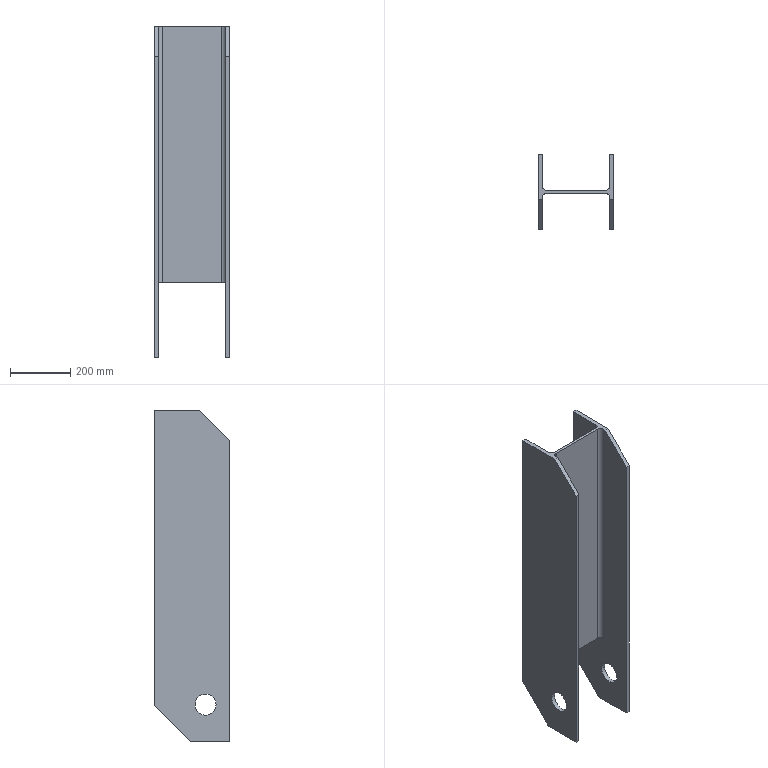Component | SolidWorks | WeldedI-beam-1_250I-beam-1 | 1 solid | 26 faces | box 250 x 250 x 1100 mm | volume 9072254 mm3 | plane 18 | cylinder 8 | commonest cylinder face diameters 70 x4 26 x4 | material Plain Carbon Steel
build123d program:
from build123d import *

# Parameters (mm, degrees)
BOSS_EXTRUDE1_DEPTH = 1100
SKETCH2_W           = 222
SKETCH2_H           = 250
CUT_EXTRUDE1_DEPTH  = 1156.422
CHAMFER1_SIZE       = 100
CHAMFER2_SIZE       = 120
SKETCH3_R           = 35
CUT_EXTRUDE2_DEPTH  = 1156.422


with BuildPart() as part:
    # Sketch1 → Boss-Extrude1 (new body)
    with BuildSketch(Plane(origin=(0, 0, 0), x_dir=(1, 0, 0), z_dir=(0, 1, 0))):
        with BuildLine():
            Line((0, 0), (250, 0))
            Line((250, 0), (250, -14))
            Line((250, -14), (142.5, -14))
            ThreePointArc((142.5, -14), (133.308, -17.808), (129.5, -27))
            Line((129.5, -27), (129.5, -223))
            ThreePointArc((129.5, -223), (133.308, -232.192), (142.5, -236))
            Line((142.5, -236), (250, -236))
            Line((250, -236), (250, -250))
            Line((250, -250), (0, -250))
            Line((0, -250), (0, -236))
            Line((0, -236), (107.5, -236))
            ThreePointArc((107.5, -236), (116.692, -232.192), (120.5, -223))
            Line((120.5, -223), (120.5, -27))
            ThreePointArc((120.5, -27), (116.692, -17.808), (107.5, -14))
            Line((107.5, -14), (0, -14))
            Line((0, -14), (0, 0))
        make_face()
    extrude(amount=BOSS_EXTRUDE1_DEPTH)

    # Sketch2 → Cut-Extrude1 (cut, through all)
    with BuildSketch(Plane.ZY):
        with Locations((125, 125)):
            Rectangle(SKETCH2_W, SKETCH2_H)
    extrude(amount=-CUT_EXTRUDE1_DEPTH, mode=Mode.SUBTRACT)

    # Chamfer1
    chamfer1_edges = [part.edges().sort_by_distance(p)[0] for p in [
        (250, 1100, 243),
        (250, 1100, 7),
    ]]
    chamfer(chamfer1_edges, length=CHAMFER1_SIZE)

    # Chamfer2
    chamfer2_edges = [part.edges().sort_by_distance(p)[0] for p in [
        (0, 0, 243),
        (0, 0, 7),
    ]]
    chamfer(chamfer2_edges, length=CHAMFER2_SIZE)

    # Sketch3 → Cut-Extrude2 (cut, through all)
    with BuildSketch(Plane.XY.offset(250)):
        with Locations((170, 123)):
            Circle(SKETCH3_R)
    extrude(amount=-CUT_EXTRUDE2_DEPTH, mode=Mode.SUBTRACT)


solid = part.part

# Placed as in the assembly
solid = solid.moved(Location((-6247.465, 2931.733, 5424.043), (90, -90, 0)))
STEP:
#1=CARTESIAN_POINT('',(-255.255,110.108,218.388));
#2=VERTEX_POINT('',#1);
#3=CARTESIAN_POINT('',(-255.255,107.352,218.388));
#4=VERTEX_POINT('',#3);
#5=CARTESIAN_POINT('',(-255.255,108.73,218.388));
#6=DIRECTION('',(-1.,-0.,0.));
#7=DIRECTION('',(0.,-1.,0.));
#8=AXIS2_PLACEMENT_3D('',#5,#6,#7);
#9=CIRCLE('',#8,1.378);
#10=EDGE_CURVE('',#2,#4,#9,.T.);
#11=ORIENTED_EDGE('',*,*,#10,.F.);
#12=CARTESIAN_POINT('',(-255.806,110.108,218.388));
#13=VERTEX_POINT('',#12);
#14=CARTESIAN_POINT('',(-245.963,110.108,218.388));
#15=DIRECTION('',(-1.,-0.,0.));
#16=VECTOR('',#15,39.37);
#17=LINE('',#14,#16);
#18=EDGE_CURVE('',#2,#13,#17,.T.);
#19=ORIENTED_EDGE('',*,*,#18,.T.);
#20=CARTESIAN_POINT('',(-255.806,107.352,218.388));
#21=VERTEX_POINT('',#20);
#22=CARTESIAN_POINT('',(-255.806,108.73,218.388));
#23=DIRECTION('',(-1.,-0.,0.));
#24=DIRECTION('',(0.,-1.,0.));
#25=AXIS2_PLACEMENT_3D('',#22,#23,#24);
#26=CIRCLE('',#25,1.378);
#27=EDGE_CURVE('',#13,#21,#26,.T.);
#28=ORIENTED_EDGE('',*,*,#27,.T.);
#29=CARTESIAN_POINT('',(-245.963,107.352,218.388));
#30=DIRECTION('',(-1.,-0.,0.));
#31=VECTOR('',#30,39.37);
#32=LINE('',#29,#31);
#33=EDGE_CURVE('',#4,#21,#32,.T.);
#34=ORIENTED_EDGE('',*,*,#33,.F.);
#35=EDGE_LOOP('',(#11,#19,#28,#34));
#36=FACE_OUTER_BOUND('',#35,.T.);
#37=CARTESIAN_POINT('',(-245.963,108.73,218.388));
#38=DIRECTION('',(-1.,-0.,0.));
#39=DIRECTION('',(0.,-1.,0.));
#40=AXIS2_PLACEMENT_3D('',#37,#38,#39);
#41=CYLINDRICAL_SURFACE('',#40,1.378);
#42=ADVANCED_FACE('',(#36),#41,.F.);
#43=CARTESIAN_POINT('',(-245.963,110.108,218.388));
#44=VERTEX_POINT('',#43);
#45=CARTESIAN_POINT('',(-245.963,107.352,218.388));
#46=VERTEX_POINT('',#45);
#47=CARTESIAN_POINT('',(-245.963,108.73,218.388));
#48=DIRECTION('',(-1.,-0.,0.));
#49=DIRECTION('',(0.,-1.,0.));
#50=AXIS2_PLACEMENT_3D('',#47,#48,#49);
#51=CIRCLE('',#50,1.378);
#52=EDGE_CURVE('',#44,#46,#51,.T.);
#53=ORIENTED_EDGE('',*,*,#52,.F.);
#54=CARTESIAN_POINT('',(-246.514,110.108,218.388));
#55=VERTEX_POINT('',#54);
#56=CARTESIAN_POINT('',(-245.963,110.108,218.388));
#57=DIRECTION('',(-1.,-0.,0.));
#58=VECTOR('',#57,39.37);
#59=LINE('',#56,#58);
#60=EDGE_CURVE('',#44,#55,#59,.T.);
#61=ORIENTED_EDGE('',*,*,#60,.T.);
#62=CARTESIAN_POINT('',(-246.514,107.352,218.388));
#63=VERTEX_POINT('',#62);
#64=CARTESIAN_POINT('',(-246.514,108.73,218.388));
#65=DIRECTION('',(1.,0.,-0.));
#66=DIRECTION('',(0.,1.,0.));
#67=AXIS2_PLACEMENT_3D('',#64,#65,#66);
#68=CIRCLE('',#67,1.378);
#69=EDGE_CURVE('',#63,#55,#68,.T.);
#70=ORIENTED_EDGE('',*,*,#69,.F.);
#71=CARTESIAN_POINT('',(-245.963,107.352,218.388));
#72=DIRECTION('',(-1.,-0.,0.));
#73=VECTOR('',#72,39.37);
#74=LINE('',#71,#73);
#75=EDGE_CURVE('',#46,#63,#74,.T.);
#76=ORIENTED_EDGE('',*,*,#75,.F.);
#77=EDGE_LOOP('',(#53,#61,#70,#76));
#78=FACE_OUTER_BOUND('',#77,.T.);
#79=CARTESIAN_POINT('',(-245.963,108.73,218.388));
#80=DIRECTION('',(-1.,-0.,0.));
#81=DIRECTION('',(0.,-1.,0.));
#82=AXIS2_PLACEMENT_3D('',#79,#80,#81);
#83=CYLINDRICAL_SURFACE('',#82,1.378);
#84=ADVANCED_FACE('',(#78),#83,.F.);
#85=CARTESIAN_POINT('',(-255.806,110.698,213.545));
#86=VERTEX_POINT('',#85);
#87=CARTESIAN_POINT('',(-255.806,105.58,213.545));
#88=VERTEX_POINT('',#87);
#89=CARTESIAN_POINT('',(-255.806,105.58,213.545));
#90=DIRECTION('',(0.,-1.,0.));
#91=VECTOR('',#90,39.37);
#92=LINE('',#89,#91);
#93=EDGE_CURVE('',#86,#88,#92,.T.);
#94=ORIENTED_EDGE('',*,*,#93,.F.);
#95=CARTESIAN_POINT('',(-255.255,110.698,213.545));
#96=VERTEX_POINT('',#95);
#97=CARTESIAN_POINT('',(-247.026,110.698,213.545));
#98=DIRECTION('',(1.,0.,-0.));
#99=VECTOR('',#98,39.37);
#100=LINE('',#97,#99);
#101=EDGE_CURVE('',#86,#96,#100,.T.);
#102=ORIENTED_EDGE('',*,*,#101,.T.);
#103=CARTESIAN_POINT('',(-255.255,105.58,213.545));
#104=VERTEX_POINT('',#103);
#105=CARTESIAN_POINT('',(-255.255,109.812,213.545));
#106=DIRECTION('',(-0.,1.,-0.));
#107=VECTOR('',#106,39.37);
#108=LINE('',#105,#107);
#109=EDGE_CURVE('',#104,#96,#108,.T.);
#110=ORIENTED_EDGE('',*,*,#109,.F.);
#111=CARTESIAN_POINT('',(-255.255,105.58,213.545));
#112=DIRECTION('',(1.,0.,-0.));
#113=VECTOR('',#112,39.37);
#114=LINE('',#111,#113);
#115=EDGE_CURVE('',#88,#104,#114,.T.);
#116=ORIENTED_EDGE('',*,*,#115,.F.);
#117=EDGE_LOOP('',(#94,#102,#110,#116));
#118=FACE_OUTER_BOUND('',#117,.T.);
#119=CARTESIAN_POINT('',(-247.026,109.812,213.545));
#120=DIRECTION('',(-0.,0.,1.));
#121=DIRECTION('',(-1.,-0.,0.));
#122=AXIS2_PLACEMENT_3D('',#119,#120,#121);
#123=PLANE('',#122);
#124=ADVANCED_FACE('',(#118),#123,.F.);
#125=CARTESIAN_POINT('',(-245.963,115.423,256.852));
#126=VERTEX_POINT('',#125);
#127=CARTESIAN_POINT('',(-245.963,115.423,218.269));
#128=VERTEX_POINT('',#127);
#129=CARTESIAN_POINT('',(-245.963,115.423,256.852));
#130=DIRECTION('',(0.,-0.,-1.));
#131=VECTOR('',#130,39.37);
#132=LINE('',#129,#131);
#133=EDGE_CURVE('',#126,#128,#132,.T.);
#134=ORIENTED_EDGE('',*,*,#133,.T.);
#135=CARTESIAN_POINT('',(-246.514,115.423,218.269));
#136=VERTEX_POINT('',#135);
#137=CARTESIAN_POINT('',(-246.514,115.423,218.269));
#138=DIRECTION('',(-1.,-0.,0.));
#139=VECTOR('',#138,39.37);
#140=LINE('',#137,#139);
#141=EDGE_CURVE('',#128,#136,#140,.T.);
#142=ORIENTED_EDGE('',*,*,#141,.T.);
#143=CARTESIAN_POINT('',(-246.514,115.423,256.852));
#144=VERTEX_POINT('',#143);
#145=CARTESIAN_POINT('',(-246.514,115.423,256.852));
#146=DIRECTION('',(0.,-0.,-1.));
#147=VECTOR('',#146,39.37);
#148=LINE('',#145,#147);
#149=EDGE_CURVE('',#144,#136,#148,.T.);
#150=ORIENTED_EDGE('',*,*,#149,.F.);
#151=CARTESIAN_POINT('',(-246.514,115.423,256.852));
#152=DIRECTION('',(-1.,-0.,0.));
#153=VECTOR('',#152,39.37);
#154=LINE('',#151,#153);
#155=EDGE_CURVE('',#126,#144,#154,.T.);
#156=ORIENTED_EDGE('',*,*,#155,.F.);
#157=EDGE_LOOP('',(#134,#142,#150,#156));
#158=FACE_OUTER_BOUND('',#157,.T.);
#159=CARTESIAN_POINT('',(-246.514,115.423,256.852));
#160=DIRECTION('',(0.,-1.,0.));
#161=DIRECTION('',(1.,0.,-0.));
#162=AXIS2_PLACEMENT_3D('',#159,#160,#161);
#163=PLANE('',#162);
#164=ADVANCED_FACE('',(#158),#163,.F.);
#165=CARTESIAN_POINT('',(-246.514,111.19,256.852));
#166=VERTEX_POINT('',#165);
#167=CARTESIAN_POINT('',(-246.514,111.19,223.388));
#168=VERTEX_POINT('',#167);
#169=CARTESIAN_POINT('',(-246.514,111.19,256.852));
#170=DIRECTION('',(0.,-0.,-1.));
#171=VECTOR('',#170,39.37);
#172=LINE('',#169,#171);
#173=EDGE_CURVE('',#166,#168,#172,.T.);
#174=ORIENTED_EDGE('',*,*,#173,.T.);
#175=CARTESIAN_POINT('',(-247.026,110.678,223.388));
#176=VERTEX_POINT('',#175);
#177=CARTESIAN_POINT('',(-247.026,111.19,223.388));
#178=DIRECTION('',(-0.,-0.,-1.));
#179=DIRECTION('',(-1.,0.,0.));
#180=AXIS2_PLACEMENT_3D('',#177,#178,#179);
#181=CIRCLE('',#180,0.5118);
#182=EDGE_CURVE('',#168,#176,#181,.T.);
#183=ORIENTED_EDGE('',*,*,#182,.T.);
#184=CARTESIAN_POINT('',(-247.026,110.678,256.852));
#185=VERTEX_POINT('',#184);
#186=CARTESIAN_POINT('',(-247.026,110.678,256.852));
#187=DIRECTION('',(0.,-0.,-1.));
#188=VECTOR('',#187,39.37);
#189=LINE('',#186,#188);
#190=EDGE_CURVE('',#185,#176,#189,.T.);
#191=ORIENTED_EDGE('',*,*,#190,.F.);
#192=CARTESIAN_POINT('',(-247.026,111.19,256.852));
#193=DIRECTION('',(0.,-0.,-1.));
#194=DIRECTION('',(1.,0.,0.));
#195=AXIS2_PLACEMENT_3D('',#192,#193,#194);
#196=CIRCLE('',#195,0.5118);
#197=EDGE_CURVE('',#166,#185,#196,.T.);
#198=ORIENTED_EDGE('',*,*,#197,.F.);
#199=EDGE_LOOP('',(#174,#183,#191,#198));
#200=FACE_OUTER_BOUND('',#199,.T.);
#201=CARTESIAN_POINT('',(-247.026,111.19,256.852));
#202=DIRECTION('',(0.,-0.,-1.));
#203=DIRECTION('',(1.,0.,0.));
#204=AXIS2_PLACEMENT_3D('',#201,#202,#203);
#205=CYLINDRICAL_SURFACE('',#204,0.5118);
#206=ADVANCED_FACE('',(#200),#205,.F.);
#207=ORIENTED_EDGE('',*,*,#190,.T.);
#208=CARTESIAN_POINT('',(-254.743,110.678,223.388));
#209=VERTEX_POINT('',#208);
#210=CARTESIAN_POINT('',(-254.743,110.678,223.388));
#211=DIRECTION('',(-1.,-0.,0.));
#212=VECTOR('',#211,39.37);
#213=LINE('',#210,#212);
#214=EDGE_CURVE('',#176,#209,#213,.T.);
#215=ORIENTED_EDGE('',*,*,#214,.T.);
#216=CARTESIAN_POINT('',(-254.743,110.678,256.852));
#217=VERTEX_POINT('',#216);
#218=CARTESIAN_POINT('',(-254.743,110.678,256.852));
#219=DIRECTION('',(0.,-0.,-1.));
#220=VECTOR('',#219,39.37);
#221=LINE('',#218,#220);
#222=EDGE_CURVE('',#217,#209,#221,.T.);
#223=ORIENTED_EDGE('',*,*,#222,.F.);
#224=CARTESIAN_POINT('',(-254.743,110.678,256.852));
#225=DIRECTION('',(-1.,-0.,0.));
#226=VECTOR('',#225,39.37);
#227=LINE('',#224,#226);
#228=EDGE_CURVE('',#185,#217,#227,.T.);
#229=ORIENTED_EDGE('',*,*,#228,.F.);
#230=EDGE_LOOP('',(#207,#215,#223,#229));
#231=FACE_OUTER_BOUND('',#230,.T.);
#232=CARTESIAN_POINT('',(-254.743,110.678,256.852));
#233=DIRECTION('',(0.,-1.,0.));
#234=DIRECTION('',(1.,0.,-0.));
#235=AXIS2_PLACEMENT_3D('',#232,#233,#234);
#236=PLANE('',#235);
#237=ADVANCED_FACE('',(#231),#236,.F.);
#238=ORIENTED_EDGE('',*,*,#222,.T.);
#239=CARTESIAN_POINT('',(-255.255,111.19,223.388));
#240=VERTEX_POINT('',#239);
#241=CARTESIAN_POINT('',(-254.743,111.19,223.388));
#242=DIRECTION('',(-0.,-0.,-1.));
#243=DIRECTION('',(-1.,-0.,0.));
#244=AXIS2_PLACEMENT_3D('',#241,#242,#243);
#245=CIRCLE('',#244,0.5118);
#246=EDGE_CURVE('',#209,#240,#245,.T.);
#247=ORIENTED_EDGE('',*,*,#246,.T.);
#248=CARTESIAN_POINT('',(-255.255,111.19,256.852));
#249=VERTEX_POINT('',#248);
#250=CARTESIAN_POINT('',(-255.255,111.19,256.852));
#251=DIRECTION('',(0.,-0.,-1.));
#252=VECTOR('',#251,39.37);
#253=LINE('',#250,#252);
#254=EDGE_CURVE('',#249,#240,#253,.T.);
#255=ORIENTED_EDGE('',*,*,#254,.F.);
#256=CARTESIAN_POINT('',(-254.743,111.19,256.852));
#257=DIRECTION('',(0.,-0.,-1.));
#258=DIRECTION('',(-1.,0.,0.));
#259=AXIS2_PLACEMENT_3D('',#256,#257,#258);
#260=CIRCLE('',#259,0.5118);
#261=EDGE_CURVE('',#217,#249,#260,.T.);
#262=ORIENTED_EDGE('',*,*,#261,.F.);
#263=EDGE_LOOP('',(#238,#247,#255,#262));
#264=FACE_OUTER_BOUND('',#263,.T.);
#265=CARTESIAN_POINT('',(-254.743,111.19,256.852));
#266=DIRECTION('',(0.,-0.,-1.));
#267=DIRECTION('',(1.,0.,0.));
#268=AXIS2_PLACEMENT_3D('',#265,#266,#267);
#269=CYLINDRICAL_SURFACE('',#268,0.5118);
#270=ADVANCED_FACE('',(#264),#269,.F.);
#271=CARTESIAN_POINT('',(-255.255,115.423,256.852));
#272=VERTEX_POINT('',#271);
#273=CARTESIAN_POINT('',(-255.255,115.423,218.269));
#274=VERTEX_POINT('',#273);
#275=CARTESIAN_POINT('',(-255.255,115.423,256.852));
#276=DIRECTION('',(0.,-0.,-1.));
#277=VECTOR('',#276,39.37);
#278=LINE('',#275,#277);
#279=EDGE_CURVE('',#272,#274,#278,.T.);
#280=ORIENTED_EDGE('',*,*,#279,.T.);
#281=CARTESIAN_POINT('',(-255.806,115.423,218.269));
#282=VERTEX_POINT('',#281);
#283=CARTESIAN_POINT('',(-255.806,115.423,218.269));
#284=DIRECTION('',(-1.,-0.,0.));
#285=VECTOR('',#284,39.37);
#286=LINE('',#283,#285);
#287=EDGE_CURVE('',#274,#282,#286,.T.);
#288=ORIENTED_EDGE('',*,*,#287,.T.);
#289=CARTESIAN_POINT('',(-255.806,115.423,256.852));
#290=VERTEX_POINT('',#289);
#291=CARTESIAN_POINT('',(-255.806,115.423,256.852));
#292=DIRECTION('',(0.,-0.,-1.));
#293=VECTOR('',#292,39.37);
#294=LINE('',#291,#293);
#295=EDGE_CURVE('',#290,#282,#294,.T.);
#296=ORIENTED_EDGE('',*,*,#295,.F.);
#297=CARTESIAN_POINT('',(-255.806,115.423,256.852));
#298=DIRECTION('',(-1.,-0.,0.));
#299=VECTOR('',#298,39.37);
#300=LINE('',#297,#299);
#301=EDGE_CURVE('',#272,#290,#300,.T.);
#302=ORIENTED_EDGE('',*,*,#301,.F.);
#303=EDGE_LOOP('',(#280,#288,#296,#302));
#304=FACE_OUTER_BOUND('',#303,.T.);
#305=CARTESIAN_POINT('',(-255.806,115.423,256.852));
#306=DIRECTION('',(0.,-1.,0.));
#307=DIRECTION('',(1.,0.,-0.));
#308=AXIS2_PLACEMENT_3D('',#305,#306,#307);
#309=PLANE('',#308);
#310=ADVANCED_FACE('',(#304),#309,.F.);
#311=CARTESIAN_POINT('',(-255.806,108.73,218.388));
#312=DIRECTION('',(-1.,-0.,0.));
#313=DIRECTION('',(0.,-1.,0.));
#314=AXIS2_PLACEMENT_3D('',#311,#312,#313);
#315=CIRCLE('',#314,1.378);
#316=EDGE_CURVE('',#21,#13,#315,.T.);
#317=ORIENTED_EDGE('',*,*,#316,.F.);
#318=ORIENTED_EDGE('',*,*,#27,.F.);
#319=EDGE_LOOP('',(#317,#318));
#320=FACE_BOUND('',#319,.T.);
#321=ORIENTED_EDGE('',*,*,#295,.T.);
#322=CARTESIAN_POINT('',(-255.806,115.423,218.269));
#323=DIRECTION('',(0.,-0.7071,-0.7071));
#324=VECTOR('',#323,39.37);
#325=LINE('',#322,#324);
#326=EDGE_CURVE('',#282,#86,#325,.T.);
#327=ORIENTED_EDGE('',*,*,#326,.T.);
#328=ORIENTED_EDGE('',*,*,#93,.T.);
#329=CARTESIAN_POINT('',(-255.806,105.58,252.915));
#330=VERTEX_POINT('',#329);
#331=CARTESIAN_POINT('',(-255.806,105.58,256.852));
#332=DIRECTION('',(0.,-0.,-1.));
#333=VECTOR('',#332,39.37);
#334=LINE('',#331,#333);
#335=EDGE_CURVE('',#330,#88,#334,.T.);
#336=ORIENTED_EDGE('',*,*,#335,.F.);
#337=CARTESIAN_POINT('',(-255.806,109.517,256.852));
#338=VERTEX_POINT('',#337);
#339=CARTESIAN_POINT('',(-255.806,109.517,256.852));
#340=DIRECTION('',(-0.,0.7071,0.7071));
#341=VECTOR('',#340,39.37);
#342=LINE('',#339,#341);
#343=EDGE_CURVE('',#330,#338,#342,.T.);
#344=ORIENTED_EDGE('',*,*,#343,.T.);
#345=CARTESIAN_POINT('',(-255.806,105.58,256.852));
#346=DIRECTION('',(0.,-1.,0.));
#347=VECTOR('',#346,39.37);
#348=LINE('',#345,#347);
#349=EDGE_CURVE('',#290,#338,#348,.T.);
#350=ORIENTED_EDGE('',*,*,#349,.F.);
#351=EDGE_LOOP('',(#321,#327,#328,#336,#344,#350));
#352=FACE_OUTER_BOUND('',#351,.T.);
#353=CARTESIAN_POINT('',(-255.806,105.58,256.852));
#354=DIRECTION('',(1.,0.,-0.));
#355=DIRECTION('',(-0.,1.,-0.));
#356=AXIS2_PLACEMENT_3D('',#353,#354,#355);
#357=PLANE('',#356);
#358=ADVANCED_FACE('',(#320,#352),#357,.F.);
#359=CARTESIAN_POINT('',(-255.255,105.58,252.915));
#360=VERTEX_POINT('',#359);
#361=CARTESIAN_POINT('',(-255.255,105.58,256.852));
#362=DIRECTION('',(0.,-0.,-1.));
#363=VECTOR('',#362,39.37);
#364=LINE('',#361,#363);
#365=EDGE_CURVE('',#360,#104,#364,.T.);
#366=ORIENTED_EDGE('',*,*,#365,.F.);
#367=CARTESIAN_POINT('',(-255.806,105.58,252.915));
#368=DIRECTION('',(-1.,-0.,0.));
#369=VECTOR('',#368,39.37);
#370=LINE('',#367,#369);
#371=EDGE_CURVE('',#360,#330,#370,.T.);
#372=ORIENTED_EDGE('',*,*,#371,.T.);
#373=ORIENTED_EDGE('',*,*,#335,.T.);
#374=ORIENTED_EDGE('',*,*,#115,.T.);
#375=EDGE_LOOP('',(#366,#372,#373,#374));
#376=FACE_OUTER_BOUND('',#375,.T.);
#377=CARTESIAN_POINT('',(-255.255,105.58,256.852));
#378=DIRECTION('',(-0.,1.,-0.));
#379=DIRECTION('',(-1.,-0.,0.));
#380=AXIS2_PLACEMENT_3D('',#377,#378,#379);
#381=PLANE('',#380);
#382=ADVANCED_FACE('',(#376),#381,.F.);
#383=CARTESIAN_POINT('',(-255.255,108.73,218.388));
#384=DIRECTION('',(-1.,-0.,0.));
#385=DIRECTION('',(0.,-1.,0.));
#386=AXIS2_PLACEMENT_3D('',#383,#384,#385);
#387=CIRCLE('',#386,1.378);
#388=EDGE_CURVE('',#4,#2,#387,.T.);
#389=ORIENTED_EDGE('',*,*,#388,.T.);
#390=ORIENTED_EDGE('',*,*,#10,.T.);
#391=EDGE_LOOP('',(#389,#390));
#392=FACE_BOUND('',#391,.T.);
#393=ORIENTED_EDGE('',*,*,#109,.T.);
#394=CARTESIAN_POINT('',(-255.255,115.423,218.269));
#395=DIRECTION('',(-0.,0.7071,0.7071));
#396=VECTOR('',#395,39.37);
#397=LINE('',#394,#396);
#398=EDGE_CURVE('',#96,#274,#397,.T.);
#399=ORIENTED_EDGE('',*,*,#398,.T.);
#400=ORIENTED_EDGE('',*,*,#279,.F.);
#401=CARTESIAN_POINT('',(-255.255,115.423,256.852));
#402=DIRECTION('',(-0.,1.,-0.));
#403=VECTOR('',#402,39.37);
#404=LINE('',#401,#403);
#405=EDGE_CURVE('',#249,#272,#404,.T.);
#406=ORIENTED_EDGE('',*,*,#405,.F.);
#407=ORIENTED_EDGE('',*,*,#254,.T.);
#408=CARTESIAN_POINT('',(-255.255,109.812,223.388));
#409=VERTEX_POINT('',#408);
#410=CARTESIAN_POINT('',(-255.255,105.58,223.388));
#411=DIRECTION('',(-0.,1.,-0.));
#412=VECTOR('',#411,39.37);
#413=LINE('',#410,#412);
#414=EDGE_CURVE('',#409,#240,#413,.T.);
#415=ORIENTED_EDGE('',*,*,#414,.F.);
#416=CARTESIAN_POINT('',(-255.255,109.812,256.852));
#417=VERTEX_POINT('',#416);
#418=CARTESIAN_POINT('',(-255.255,109.812,256.852));
#419=DIRECTION('',(0.,-0.,-1.));
#420=VECTOR('',#419,39.37);
#421=LINE('',#418,#420);
#422=EDGE_CURVE('',#417,#409,#421,.T.);
#423=ORIENTED_EDGE('',*,*,#422,.F.);
#424=CARTESIAN_POINT('',(-255.255,109.517,256.852));
#425=VERTEX_POINT('',#424);
#426=CARTESIAN_POINT('',(-255.255,109.812,256.852));
#427=DIRECTION('',(-0.,1.,-0.));
#428=VECTOR('',#427,39.37);
#429=LINE('',#426,#428);
#430=EDGE_CURVE('',#425,#417,#429,.T.);
#431=ORIENTED_EDGE('',*,*,#430,.F.);
#432=CARTESIAN_POINT('',(-255.255,109.517,256.852));
#433=DIRECTION('',(0.,-0.7071,-0.7071));
#434=VECTOR('',#433,39.37);
#435=LINE('',#432,#434);
#436=EDGE_CURVE('',#425,#360,#435,.T.);
#437=ORIENTED_EDGE('',*,*,#436,.T.);
#438=ORIENTED_EDGE('',*,*,#365,.T.);
#439=EDGE_LOOP('',(#393,#399,#400,#406,#407,#415,#423,#431,#437,#438));
#440=FACE_OUTER_BOUND('',#439,.T.);
#441=CARTESIAN_POINT('',(-255.255,109.812,256.852));
#442=DIRECTION('',(-1.,-0.,0.));
#443=DIRECTION('',(0.,-1.,0.));
#444=AXIS2_PLACEMENT_3D('',#441,#442,#443);
#445=PLANE('',#444);
#446=ADVANCED_FACE('',(#392,#440),#445,.F.);
#447=ORIENTED_EDGE('',*,*,#422,.T.);
#448=CARTESIAN_POINT('',(-254.743,110.324,223.388));
#449=VERTEX_POINT('',#448);
#450=CARTESIAN_POINT('',(-254.743,109.812,223.388));
#451=DIRECTION('',(-0.,-0.,-1.));
#452=DIRECTION('',(-1.,0.,0.));
#453=AXIS2_PLACEMENT_3D('',#450,#451,#452);
#454=CIRCLE('',#453,0.5118);
#455=EDGE_CURVE('',#409,#449,#454,.T.);
#456=ORIENTED_EDGE('',*,*,#455,.T.);
#457=CARTESIAN_POINT('',(-254.743,110.324,256.852));
#458=VERTEX_POINT('',#457);
#459=CARTESIAN_POINT('',(-254.743,110.324,256.852));
#460=DIRECTION('',(0.,-0.,-1.));
#461=VECTOR('',#460,39.37);
#462=LINE('',#459,#461);
#463=EDGE_CURVE('',#458,#449,#462,.T.);
#464=ORIENTED_EDGE('',*,*,#463,.F.);
#465=CARTESIAN_POINT('',(-254.743,109.812,256.852));
#466=DIRECTION('',(0.,-0.,-1.));
#467=DIRECTION('',(-1.,0.,0.));
#468=AXIS2_PLACEMENT_3D('',#465,#466,#467);
#469=CIRCLE('',#468,0.5118);
#470=EDGE_CURVE('',#417,#458,#469,.T.);
#471=ORIENTED_EDGE('',*,*,#470,.F.);
#472=EDGE_LOOP('',(#447,#456,#464,#471));
#473=FACE_OUTER_BOUND('',#472,.T.);
#474=CARTESIAN_POINT('',(-254.743,109.812,256.852));
#475=DIRECTION('',(0.,-0.,-1.));
#476=DIRECTION('',(1.,0.,0.));
#477=AXIS2_PLACEMENT_3D('',#474,#475,#476);
#478=CYLINDRICAL_SURFACE('',#477,0.5118);
#479=ADVANCED_FACE('',(#473),#478,.F.);
#480=ORIENTED_EDGE('',*,*,#463,.T.);
#481=CARTESIAN_POINT('',(-247.026,110.324,223.388));
#482=VERTEX_POINT('',#481);
#483=CARTESIAN_POINT('',(-247.026,110.324,223.388));
#484=DIRECTION('',(1.,0.,-0.));
#485=VECTOR('',#484,39.37);
#486=LINE('',#483,#485);
#487=EDGE_CURVE('',#449,#482,#486,.T.);
#488=ORIENTED_EDGE('',*,*,#487,.T.);
#489=CARTESIAN_POINT('',(-247.026,110.324,256.852));
#490=VERTEX_POINT('',#489);
#491=CARTESIAN_POINT('',(-247.026,110.324,256.852));
#492=DIRECTION('',(0.,-0.,-1.));
#493=VECTOR('',#492,39.37);
#494=LINE('',#491,#493);
#495=EDGE_CURVE('',#490,#482,#494,.T.);
#496=ORIENTED_EDGE('',*,*,#495,.F.);
#497=CARTESIAN_POINT('',(-247.026,110.324,256.852));
#498=DIRECTION('',(1.,0.,-0.));
#499=VECTOR('',#498,39.37);
#500=LINE('',#497,#499);
#501=EDGE_CURVE('',#458,#490,#500,.T.);
#502=ORIENTED_EDGE('',*,*,#501,.F.);
#503=EDGE_LOOP('',(#480,#488,#496,#502));
#504=FACE_OUTER_BOUND('',#503,.T.);
#505=CARTESIAN_POINT('',(-247.026,110.324,256.852));
#506=DIRECTION('',(-0.,1.,-0.));
#507=DIRECTION('',(-1.,-0.,0.));
#508=AXIS2_PLACEMENT_3D('',#505,#506,#507);
#509=PLANE('',#508);
#510=ADVANCED_FACE('',(#504),#509,.F.);
#511=ORIENTED_EDGE('',*,*,#495,.T.);
#512=CARTESIAN_POINT('',(-246.514,109.812,223.388));
#513=VERTEX_POINT('',#512);
#514=CARTESIAN_POINT('',(-247.026,109.812,223.388));
#515=DIRECTION('',(-0.,-0.,-1.));
#516=DIRECTION('',(-1.,0.,0.));
#517=AXIS2_PLACEMENT_3D('',#514,#515,#516);
#518=CIRCLE('',#517,0.5118);
#519=EDGE_CURVE('',#482,#513,#518,.T.);
#520=ORIENTED_EDGE('',*,*,#519,.T.);
#521=CARTESIAN_POINT('',(-246.514,109.812,256.852));
#522=VERTEX_POINT('',#521);
#523=CARTESIAN_POINT('',(-246.514,109.812,256.852));
#524=DIRECTION('',(0.,-0.,-1.));
#525=VECTOR('',#524,39.37);
#526=LINE('',#523,#525);
#527=EDGE_CURVE('',#522,#513,#526,.T.);
#528=ORIENTED_EDGE('',*,*,#527,.F.);
#529=CARTESIAN_POINT('',(-247.026,109.812,256.852));
#530=DIRECTION('',(0.,-0.,-1.));
#531=DIRECTION('',(-1.,0.,0.));
#532=AXIS2_PLACEMENT_3D('',#529,#530,#531);
#533=CIRCLE('',#532,0.5118);
#534=EDGE_CURVE('',#490,#522,#533,.T.);
#535=ORIENTED_EDGE('',*,*,#534,.F.);
#536=EDGE_LOOP('',(#511,#520,#528,#535));
#537=FACE_OUTER_BOUND('',#536,.T.);
#538=CARTESIAN_POINT('',(-247.026,109.812,256.852));
#539=DIRECTION('',(0.,-0.,-1.));
#540=DIRECTION('',(1.,0.,0.));
#541=AXIS2_PLACEMENT_3D('',#538,#539,#540);
#542=CYLINDRICAL_SURFACE('',#541,0.5118);
#543=ADVANCED_FACE('',(#537),#542,.F.);
#544=ORIENTED_EDGE('',*,*,#69,.T.);
#545=CARTESIAN_POINT('',(-246.514,108.73,218.388));
#546=DIRECTION('',(1.,0.,-0.));
#547=DIRECTION('',(0.,1.,0.));
#548=AXIS2_PLACEMENT_3D('',#545,#546,#547);
#549=CIRCLE('',#548,1.378);
#550=EDGE_CURVE('',#55,#63,#549,.T.);
#551=ORIENTED_EDGE('',*,*,#550,.T.);
#552=EDGE_LOOP('',(#544,#551));
#553=FACE_BOUND('',#552,.T.);
#554=ORIENTED_EDGE('',*,*,#149,.T.);
#555=CARTESIAN_POINT('',(-246.514,110.698,213.545));
#556=VERTEX_POINT('',#555);
#557=CARTESIAN_POINT('',(-246.514,115.423,218.269));
#558=DIRECTION('',(0.,-0.7071,-0.7071));
#559=VECTOR('',#558,39.37);
#560=LINE('',#557,#559);
#561=EDGE_CURVE('',#136,#556,#560,.T.);
#562=ORIENTED_EDGE('',*,*,#561,.T.);
#563=CARTESIAN_POINT('',(-246.514,105.58,213.545));
#564=VERTEX_POINT('',#563);
#565=CARTESIAN_POINT('',(-246.514,105.58,213.545));
#566=DIRECTION('',(0.,-1.,0.));
#567=VECTOR('',#566,39.37);
#568=LINE('',#565,#567);
#569=EDGE_CURVE('',#556,#564,#568,.T.);
#570=ORIENTED_EDGE('',*,*,#569,.T.);
#571=CARTESIAN_POINT('',(-246.514,105.58,252.915));
#572=VERTEX_POINT('',#571);
#573=CARTESIAN_POINT('',(-246.514,105.58,256.852));
#574=DIRECTION('',(0.,-0.,-1.));
#575=VECTOR('',#574,39.37);
#576=LINE('',#573,#575);
#577=EDGE_CURVE('',#572,#564,#576,.T.);
#578=ORIENTED_EDGE('',*,*,#577,.F.);
#579=CARTESIAN_POINT('',(-246.514,109.517,256.852));
#580=VERTEX_POINT('',#579);
#581=CARTESIAN_POINT('',(-246.514,109.517,256.852));
#582=DIRECTION('',(-0.,0.7071,0.7071));
#583=VECTOR('',#582,39.37);
#584=LINE('',#581,#583);
#585=EDGE_CURVE('',#572,#580,#584,.T.);
#586=ORIENTED_EDGE('',*,*,#585,.T.);
#587=CARTESIAN_POINT('',(-246.514,105.58,256.852));
#588=DIRECTION('',(0.,-1.,0.));
#589=VECTOR('',#588,39.37);
#590=LINE('',#587,#589);
#591=EDGE_CURVE('',#522,#580,#590,.T.);
#592=ORIENTED_EDGE('',*,*,#591,.F.);
#593=ORIENTED_EDGE('',*,*,#527,.T.);
#594=CARTESIAN_POINT('',(-246.514,105.58,223.388));
#595=DIRECTION('',(-0.,1.,-0.));
#596=VECTOR('',#595,39.37);
#597=LINE('',#594,#596);
#598=EDGE_CURVE('',#513,#168,#597,.T.);
#599=ORIENTED_EDGE('',*,*,#598,.T.);
#600=ORIENTED_EDGE('',*,*,#173,.F.);
#601=CARTESIAN_POINT('',(-246.514,111.19,256.852));
#602=DIRECTION('',(0.,-1.,0.));
#603=VECTOR('',#602,39.37);
#604=LINE('',#601,#603);
#605=EDGE_CURVE('',#144,#166,#604,.T.);
#606=ORIENTED_EDGE('',*,*,#605,.F.);
#607=EDGE_LOOP('',(#554,#562,#570,#578,#586,#592,#593,#599,#600,#606));
#608=FACE_OUTER_BOUND('',#607,.T.);
#609=CARTESIAN_POINT('',(-246.514,105.58,256.852));
#610=DIRECTION('',(1.,0.,-0.));
#611=DIRECTION('',(-0.,1.,-0.));
#612=AXIS2_PLACEMENT_3D('',#609,#610,#611);
#613=PLANE('',#612);
#614=ADVANCED_FACE('',(#553,#608),#613,.F.);
#615=CARTESIAN_POINT('',(-245.963,105.58,252.915));
#616=VERTEX_POINT('',#615);
#617=CARTESIAN_POINT('',(-245.963,105.58,213.545));
#618=VERTEX_POINT('',#617);
#619=CARTESIAN_POINT('',(-245.963,105.58,256.852));
#620=DIRECTION('',(0.,-0.,-1.));
#621=VECTOR('',#620,39.37);
#622=LINE('',#619,#621);
#623=EDGE_CURVE('',#616,#618,#622,.T.);
#624=ORIENTED_EDGE('',*,*,#623,.F.);
#625=CARTESIAN_POINT('',(-246.514,105.58,252.915));
#626=DIRECTION('',(-1.,-0.,0.));
#627=VECTOR('',#626,39.37);
#628=LINE('',#625,#627);
#629=EDGE_CURVE('',#616,#572,#628,.T.);
#630=ORIENTED_EDGE('',*,*,#629,.T.);
#631=ORIENTED_EDGE('',*,*,#577,.T.);
#632=CARTESIAN_POINT('',(-245.963,105.58,213.545));
#633=DIRECTION('',(1.,0.,-0.));
#634=VECTOR('',#633,39.37);
#635=LINE('',#632,#634);
#636=EDGE_CURVE('',#564,#618,#635,.T.);
#637=ORIENTED_EDGE('',*,*,#636,.T.);
#638=EDGE_LOOP('',(#624,#630,#631,#637));
#639=FACE_OUTER_BOUND('',#638,.T.);
#640=CARTESIAN_POINT('',(-245.963,105.58,256.852));
#641=DIRECTION('',(-0.,1.,-0.));
#642=DIRECTION('',(-1.,-0.,0.));
#643=AXIS2_PLACEMENT_3D('',#640,#641,#642);
#644=PLANE('',#643);
#645=ADVANCED_FACE('',(#639),#644,.F.);
#646=CARTESIAN_POINT('',(-245.963,108.73,218.388));
#647=DIRECTION('',(-1.,-0.,0.));
#648=DIRECTION('',(0.,-1.,0.));
#649=AXIS2_PLACEMENT_3D('',#646,#647,#648);
#650=CIRCLE('',#649,1.378);
#651=EDGE_CURVE('',#46,#44,#650,.T.);
#652=ORIENTED_EDGE('',*,*,#651,.T.);
#653=ORIENTED_EDGE('',*,*,#52,.T.);
#654=EDGE_LOOP('',(#652,#653));
#655=FACE_BOUND('',#654,.T.);
#656=CARTESIAN_POINT('',(-245.963,110.698,213.545));
#657=VERTEX_POINT('',#656);
#658=CARTESIAN_POINT('',(-245.963,115.423,213.545));
#659=DIRECTION('',(-0.,1.,-0.));
#660=VECTOR('',#659,39.37);
#661=LINE('',#658,#660);
#662=EDGE_CURVE('',#618,#657,#661,.T.);
#663=ORIENTED_EDGE('',*,*,#662,.T.);
#664=CARTESIAN_POINT('',(-245.963,115.423,218.269));
#665=DIRECTION('',(-0.,0.7071,0.7071));
#666=VECTOR('',#665,39.37);
#667=LINE('',#664,#666);
#668=EDGE_CURVE('',#657,#128,#667,.T.);
#669=ORIENTED_EDGE('',*,*,#668,.T.);
#670=ORIENTED_EDGE('',*,*,#133,.F.);
#671=CARTESIAN_POINT('',(-245.963,109.517,256.852));
#672=VERTEX_POINT('',#671);
#673=CARTESIAN_POINT('',(-245.963,115.423,256.852));
#674=DIRECTION('',(-0.,1.,-0.));
#675=VECTOR('',#674,39.37);
#676=LINE('',#673,#675);
#677=EDGE_CURVE('',#672,#126,#676,.T.);
#678=ORIENTED_EDGE('',*,*,#677,.F.);
#679=CARTESIAN_POINT('',(-245.963,109.517,256.852));
#680=DIRECTION('',(0.,-0.7071,-0.7071));
#681=VECTOR('',#680,39.37);
#682=LINE('',#679,#681);
#683=EDGE_CURVE('',#672,#616,#682,.T.);
#684=ORIENTED_EDGE('',*,*,#683,.T.);
#685=ORIENTED_EDGE('',*,*,#623,.T.);
#686=EDGE_LOOP('',(#663,#669,#670,#678,#684,#685));
#687=FACE_OUTER_BOUND('',#686,.T.);
#688=CARTESIAN_POINT('',(-245.963,115.423,256.852));
#689=DIRECTION('',(-1.,-0.,0.));
#690=DIRECTION('',(0.,-1.,0.));
#691=AXIS2_PLACEMENT_3D('',#688,#689,#690);
#692=PLANE('',#691);
#693=ADVANCED_FACE('',(#655,#687),#692,.F.);
#694=ORIENTED_EDGE('',*,*,#591,.T.);
#695=CARTESIAN_POINT('',(-245.963,109.517,256.852));
#696=DIRECTION('',(1.,0.,-0.));
#697=VECTOR('',#696,39.37);
#698=LINE('',#695,#697);
#699=EDGE_CURVE('',#580,#672,#698,.T.);
#700=ORIENTED_EDGE('',*,*,#699,.T.);
#701=ORIENTED_EDGE('',*,*,#677,.T.);
#702=ORIENTED_EDGE('',*,*,#155,.T.);
#703=ORIENTED_EDGE('',*,*,#605,.T.);
#704=ORIENTED_EDGE('',*,*,#197,.T.);
#705=ORIENTED_EDGE('',*,*,#228,.T.);
#706=ORIENTED_EDGE('',*,*,#261,.T.);
#707=ORIENTED_EDGE('',*,*,#405,.T.);
#708=ORIENTED_EDGE('',*,*,#301,.T.);
#709=ORIENTED_EDGE('',*,*,#349,.T.);
#710=CARTESIAN_POINT('',(-255.255,109.517,256.852));
#711=DIRECTION('',(1.,0.,-0.));
#712=VECTOR('',#711,39.37);
#713=LINE('',#710,#712);
#714=EDGE_CURVE('',#338,#425,#713,.T.);
#715=ORIENTED_EDGE('',*,*,#714,.T.);
#716=ORIENTED_EDGE('',*,*,#430,.T.);
#717=ORIENTED_EDGE('',*,*,#470,.T.);
#718=ORIENTED_EDGE('',*,*,#501,.T.);
#719=ORIENTED_EDGE('',*,*,#534,.T.);
#720=EDGE_LOOP('',(#694,#700,#701,#702,#703,#704,#705,#706,#707,#708,#709,#715,#716,#717,#718,#719));
#721=FACE_OUTER_BOUND('',#720,.T.);
#722=CARTESIAN_POINT('',(-247.026,109.812,256.852));
#723=DIRECTION('',(-0.,0.,1.));
#724=DIRECTION('',(-1.,-0.,0.));
#725=AXIS2_PLACEMENT_3D('',#722,#723,#724);
#726=PLANE('',#725);
#727=ADVANCED_FACE('',(#721),#726,.T.);
#728=ORIENTED_EDGE('',*,*,#569,.F.);
#729=CARTESIAN_POINT('',(-247.026,110.698,213.545));
#730=DIRECTION('',(1.,0.,-0.));
#731=VECTOR('',#730,39.37);
#732=LINE('',#729,#731);
#733=EDGE_CURVE('',#556,#657,#732,.T.);
#734=ORIENTED_EDGE('',*,*,#733,.T.);
#735=ORIENTED_EDGE('',*,*,#662,.F.);
#736=ORIENTED_EDGE('',*,*,#636,.F.);
#737=EDGE_LOOP('',(#728,#734,#735,#736));
#738=FACE_OUTER_BOUND('',#737,.T.);
#739=CARTESIAN_POINT('',(-247.026,109.812,213.545));
#740=DIRECTION('',(-0.,0.,1.));
#741=DIRECTION('',(-1.,-0.,0.));
#742=AXIS2_PLACEMENT_3D('',#739,#740,#741);
#743=PLANE('',#742);
#744=ADVANCED_FACE('',(#738),#743,.F.);
#745=ORIENTED_EDGE('',*,*,#598,.F.);
#746=ORIENTED_EDGE('',*,*,#519,.F.);
#747=ORIENTED_EDGE('',*,*,#487,.F.);
#748=ORIENTED_EDGE('',*,*,#455,.F.);
#749=ORIENTED_EDGE('',*,*,#414,.T.);
#750=ORIENTED_EDGE('',*,*,#246,.F.);
#751=ORIENTED_EDGE('',*,*,#214,.F.);
#752=ORIENTED_EDGE('',*,*,#182,.F.);
#753=EDGE_LOOP('',(#745,#746,#747,#748,#749,#750,#751,#752));
#754=FACE_OUTER_BOUND('',#753,.T.);
#755=CARTESIAN_POINT('',(-255.255,105.58,223.388));
#756=DIRECTION('',(0.,0.,1.));
#757=DIRECTION('',(-1.,-0.,0.));
#758=AXIS2_PLACEMENT_3D('',#755,#756,#757);
#759=PLANE('',#758);
#760=ADVANCED_FACE('',(#754),#759,.F.);
#761=ORIENTED_EDGE('',*,*,#585,.F.);
#762=ORIENTED_EDGE('',*,*,#629,.F.);
#763=ORIENTED_EDGE('',*,*,#683,.F.);
#764=ORIENTED_EDGE('',*,*,#699,.F.);
#765=EDGE_LOOP('',(#761,#762,#763,#764));
#766=FACE_OUTER_BOUND('',#765,.T.);
#767=CARTESIAN_POINT('',(-247.026,109.517,256.852));
#768=DIRECTION('',(0.,-0.7071,0.7071));
#769=DIRECTION('',(-1.,-0.,0.));
#770=AXIS2_PLACEMENT_3D('',#767,#768,#769);
#771=PLANE('',#770);
#772=ADVANCED_FACE('',(#766),#771,.T.);
#773=ORIENTED_EDGE('',*,*,#343,.F.);
#774=ORIENTED_EDGE('',*,*,#371,.F.);
#775=ORIENTED_EDGE('',*,*,#436,.F.);
#776=ORIENTED_EDGE('',*,*,#714,.F.);
#777=EDGE_LOOP('',(#773,#774,#775,#776));
#778=FACE_OUTER_BOUND('',#777,.T.);
#779=CARTESIAN_POINT('',(-247.026,109.517,256.852));
#780=DIRECTION('',(0.,-0.7071,0.7071));
#781=DIRECTION('',(-1.,-0.,0.));
#782=AXIS2_PLACEMENT_3D('',#779,#780,#781);
#783=PLANE('',#782);
#784=ADVANCED_FACE('',(#778),#783,.T.);
#785=ORIENTED_EDGE('',*,*,#398,.F.);
#786=ORIENTED_EDGE('',*,*,#101,.F.);
#787=ORIENTED_EDGE('',*,*,#326,.F.);
#788=ORIENTED_EDGE('',*,*,#287,.F.);
#789=EDGE_LOOP('',(#785,#786,#787,#788));
#790=FACE_OUTER_BOUND('',#789,.T.);
#791=CARTESIAN_POINT('',(-255.806,115.423,218.269));
#792=DIRECTION('',(0.,-0.7071,0.7071));
#793=DIRECTION('',(-1.,-0.,0.));
#794=AXIS2_PLACEMENT_3D('',#791,#792,#793);
#795=PLANE('',#794);
#796=ADVANCED_FACE('',(#790),#795,.F.);
#797=ORIENTED_EDGE('',*,*,#668,.F.);
#798=ORIENTED_EDGE('',*,*,#733,.F.);
#799=ORIENTED_EDGE('',*,*,#561,.F.);
#800=ORIENTED_EDGE('',*,*,#141,.F.);
#801=EDGE_LOOP('',(#797,#798,#799,#800));
#802=FACE_OUTER_BOUND('',#801,.T.);
#803=CARTESIAN_POINT('',(-246.514,115.423,218.269));
#804=DIRECTION('',(0.,-0.7071,0.7071));
#805=DIRECTION('',(-1.,-0.,0.));
#806=AXIS2_PLACEMENT_3D('',#803,#804,#805);
#807=PLANE('',#806);
#808=ADVANCED_FACE('',(#802),#807,.F.);
#809=ORIENTED_EDGE('',*,*,#60,.F.);
#810=ORIENTED_EDGE('',*,*,#651,.F.);
#811=ORIENTED_EDGE('',*,*,#75,.T.);
#812=ORIENTED_EDGE('',*,*,#550,.F.);
#813=EDGE_LOOP('',(#809,#810,#811,#812));
#814=FACE_OUTER_BOUND('',#813,.T.);
#815=CARTESIAN_POINT('',(-245.963,108.73,218.388));
#816=DIRECTION('',(-1.,-0.,0.));
#817=DIRECTION('',(0.,-1.,0.));
#818=AXIS2_PLACEMENT_3D('',#815,#816,#817);
#819=CYLINDRICAL_SURFACE('',#818,1.378);
#820=ADVANCED_FACE('',(#814),#819,.F.);
#821=ORIENTED_EDGE('',*,*,#18,.F.);
#822=ORIENTED_EDGE('',*,*,#388,.F.);
#823=ORIENTED_EDGE('',*,*,#33,.T.);
#824=ORIENTED_EDGE('',*,*,#316,.T.);
#825=EDGE_LOOP('',(#821,#822,#823,#824));
#826=FACE_OUTER_BOUND('',#825,.T.);
#827=CARTESIAN_POINT('',(-245.963,108.73,218.388));
#828=DIRECTION('',(-1.,-0.,0.));
#829=DIRECTION('',(0.,-1.,0.));
#830=AXIS2_PLACEMENT_3D('',#827,#828,#829);
#831=CYLINDRICAL_SURFACE('',#830,1.378);
#832=ADVANCED_FACE('',(#826),#831,.F.);
#833=CLOSED_SHELL('',(#42,#84,#124,#164,#206,#237,#270,#310,#358,#382,#446,#479,#510,#543,#614,#645,#693,#727,#744,#760,#772,#784,#796,#808,#820,#832));
#834=MANIFOLD_SOLID_BREP('',#833);
#835=CARTESIAN_POINT('',(0.,0.,0.));
#836=DIRECTION('',(0.,0.,1.));
#837=DIRECTION('',(1.,0.,0.));
#838=AXIS2_PLACEMENT_3D('',#835,#836,#837);
#839=(LENGTH_UNIT()NAMED_UNIT(*)SI_UNIT($,.METRE.));
#840=LENGTH_MEASURE_WITH_UNIT(LENGTH_MEASURE(0.0254),#839);
#841=DIMENSIONAL_EXPONENTS(1.,0.,0.,0.,0.,0.,0.);
#842=(CONVERSION_BASED_UNIT('',#840)LENGTH_UNIT()NAMED_UNIT(#841));
#843=UNCERTAINTY_MEASURE_WITH_UNIT(LENGTH_MEASURE(0.00001),#842,'','');
#844=(NAMED_UNIT(*)PLANE_ANGLE_UNIT()SI_UNIT($,.RADIAN.));
#845=(NAMED_UNIT(*)SI_UNIT($,.STERADIAN.)SOLID_ANGLE_UNIT());
#846=(GEOMETRIC_REPRESENTATION_CONTEXT(3)GLOBAL_UNCERTAINTY_ASSIGNED_CONTEXT((#843))GLOBAL_UNIT_ASSIGNED_CONTEXT((#842,#844,#845))REPRESENTATION_CONTEXT('',''));
#847=ADVANCED_BREP_SHAPE_REPRESENTATION('',(#834,#838),#846);
#848=COLOUR_RGB('',0.7922,0.8196,0.9333);
#849=FILL_AREA_STYLE_COLOUR('',#848);
#850=FILL_AREA_STYLE('',(#849));
#851=SURFACE_STYLE_FILL_AREA(#850);
#852=SURFACE_SIDE_STYLE('',(#851));
#853=SURFACE_STYLE_USAGE(.BOTH.,#852);
#854=PRESENTATION_STYLE_ASSIGNMENT((#853));
#855=STYLED_ITEM('',(#854),#834);
#856=PRESENTATION_LAYER_ASSIGNMENT('','',(#855));
#857=(LENGTH_UNIT()NAMED_UNIT(*)SI_UNIT($,.METRE.));
#858=LENGTH_MEASURE_WITH_UNIT(LENGTH_MEASURE(0.0254),#857);
#859=DIMENSIONAL_EXPONENTS(1.,0.,0.,0.,0.,0.,0.);
#860=(CONVERSION_BASED_UNIT('',#858)LENGTH_UNIT()NAMED_UNIT(#859));
#861=UNCERTAINTY_MEASURE_WITH_UNIT(LENGTH_MEASURE(0.00001),#860,'','');
#862=(NAMED_UNIT(*)PLANE_ANGLE_UNIT()SI_UNIT($,.RADIAN.));
#863=(NAMED_UNIT(*)SI_UNIT($,.STERADIAN.)SOLID_ANGLE_UNIT());
#864=(GEOMETRIC_REPRESENTATION_CONTEXT(3)GLOBAL_UNCERTAINTY_ASSIGNED_CONTEXT((#861))GLOBAL_UNIT_ASSIGNED_CONTEXT((#860,#862,#863))REPRESENTATION_CONTEXT('',''));
#865=MECHANICAL_DESIGN_GEOMETRIC_PRESENTATION_REPRESENTATION('',(#855),#864);